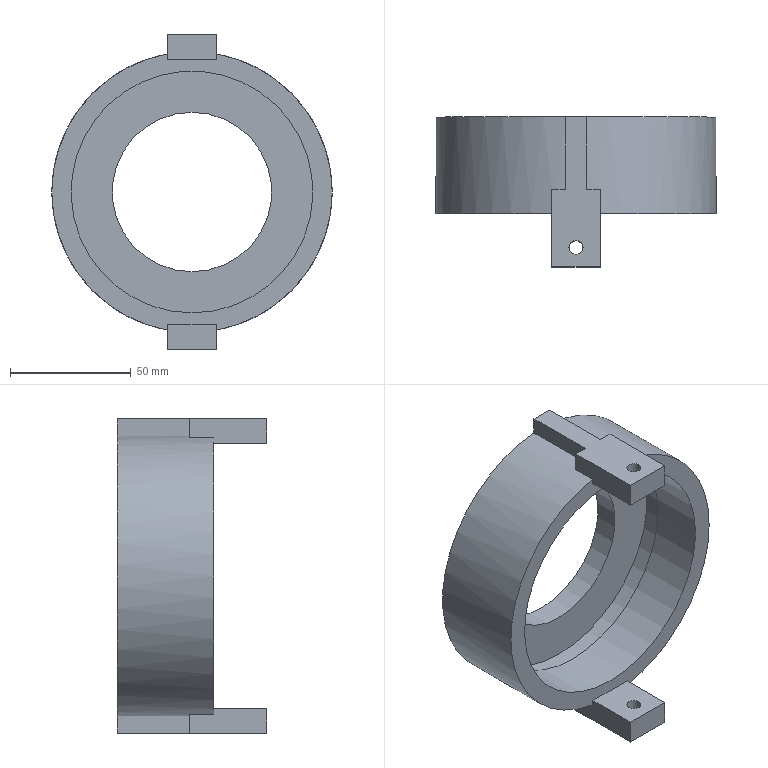Component | NX | CAP_NUT | 1 solid | 29 faces | volume 164074 mm3 | plane 22 | cylinder 7 | commonest cylinder face diameters 116 x2 5.795 x2 100 x1 103 x1 66 x1